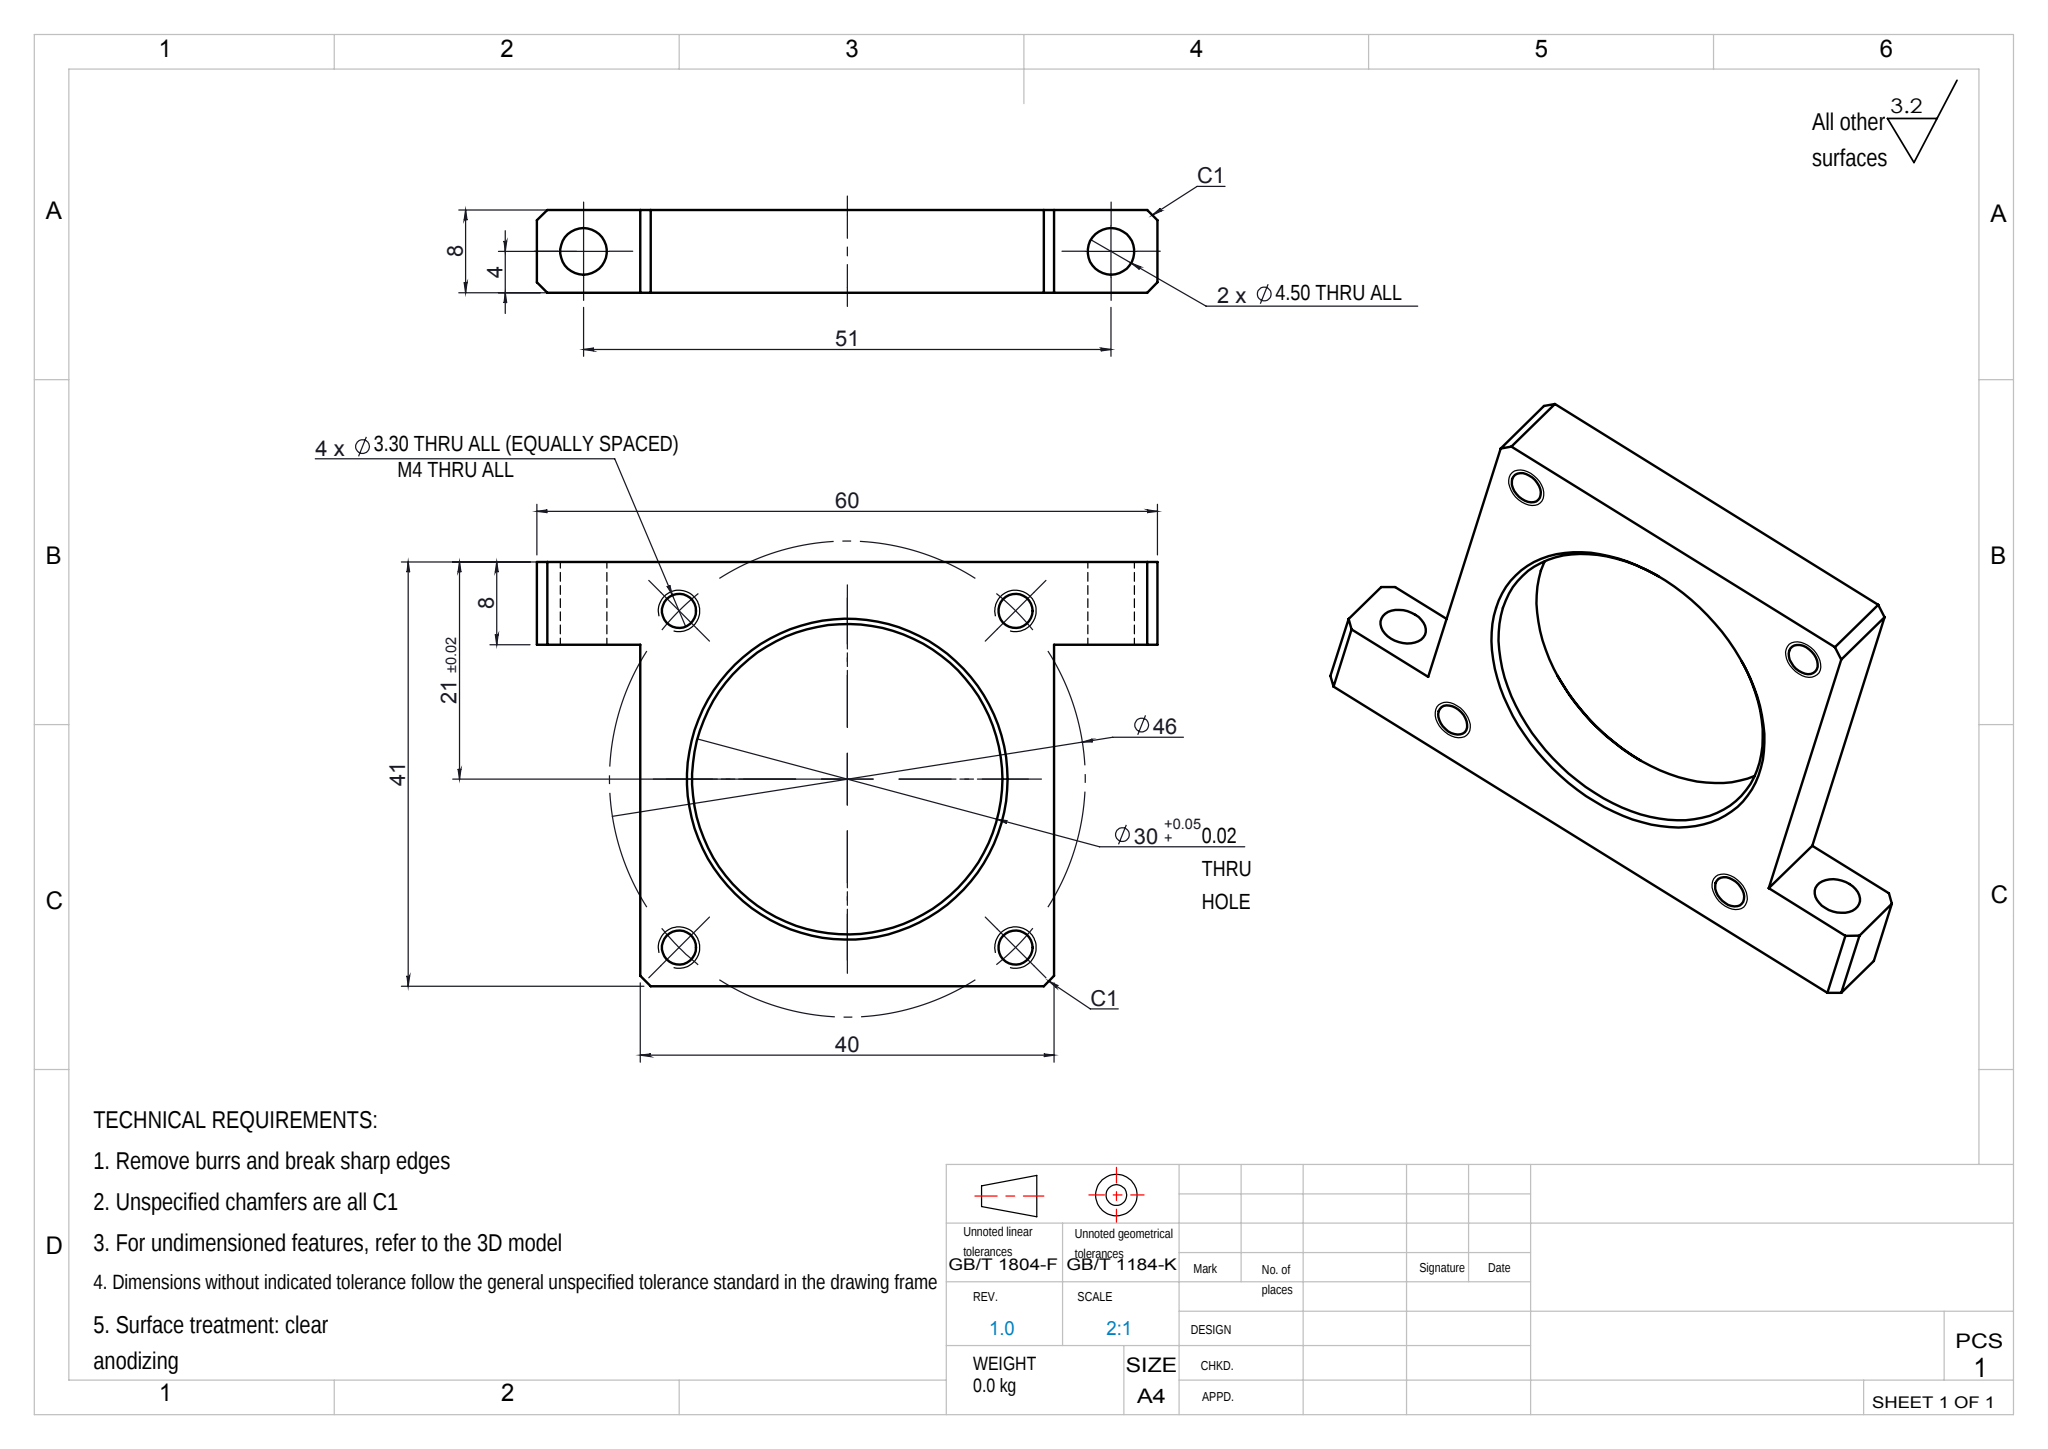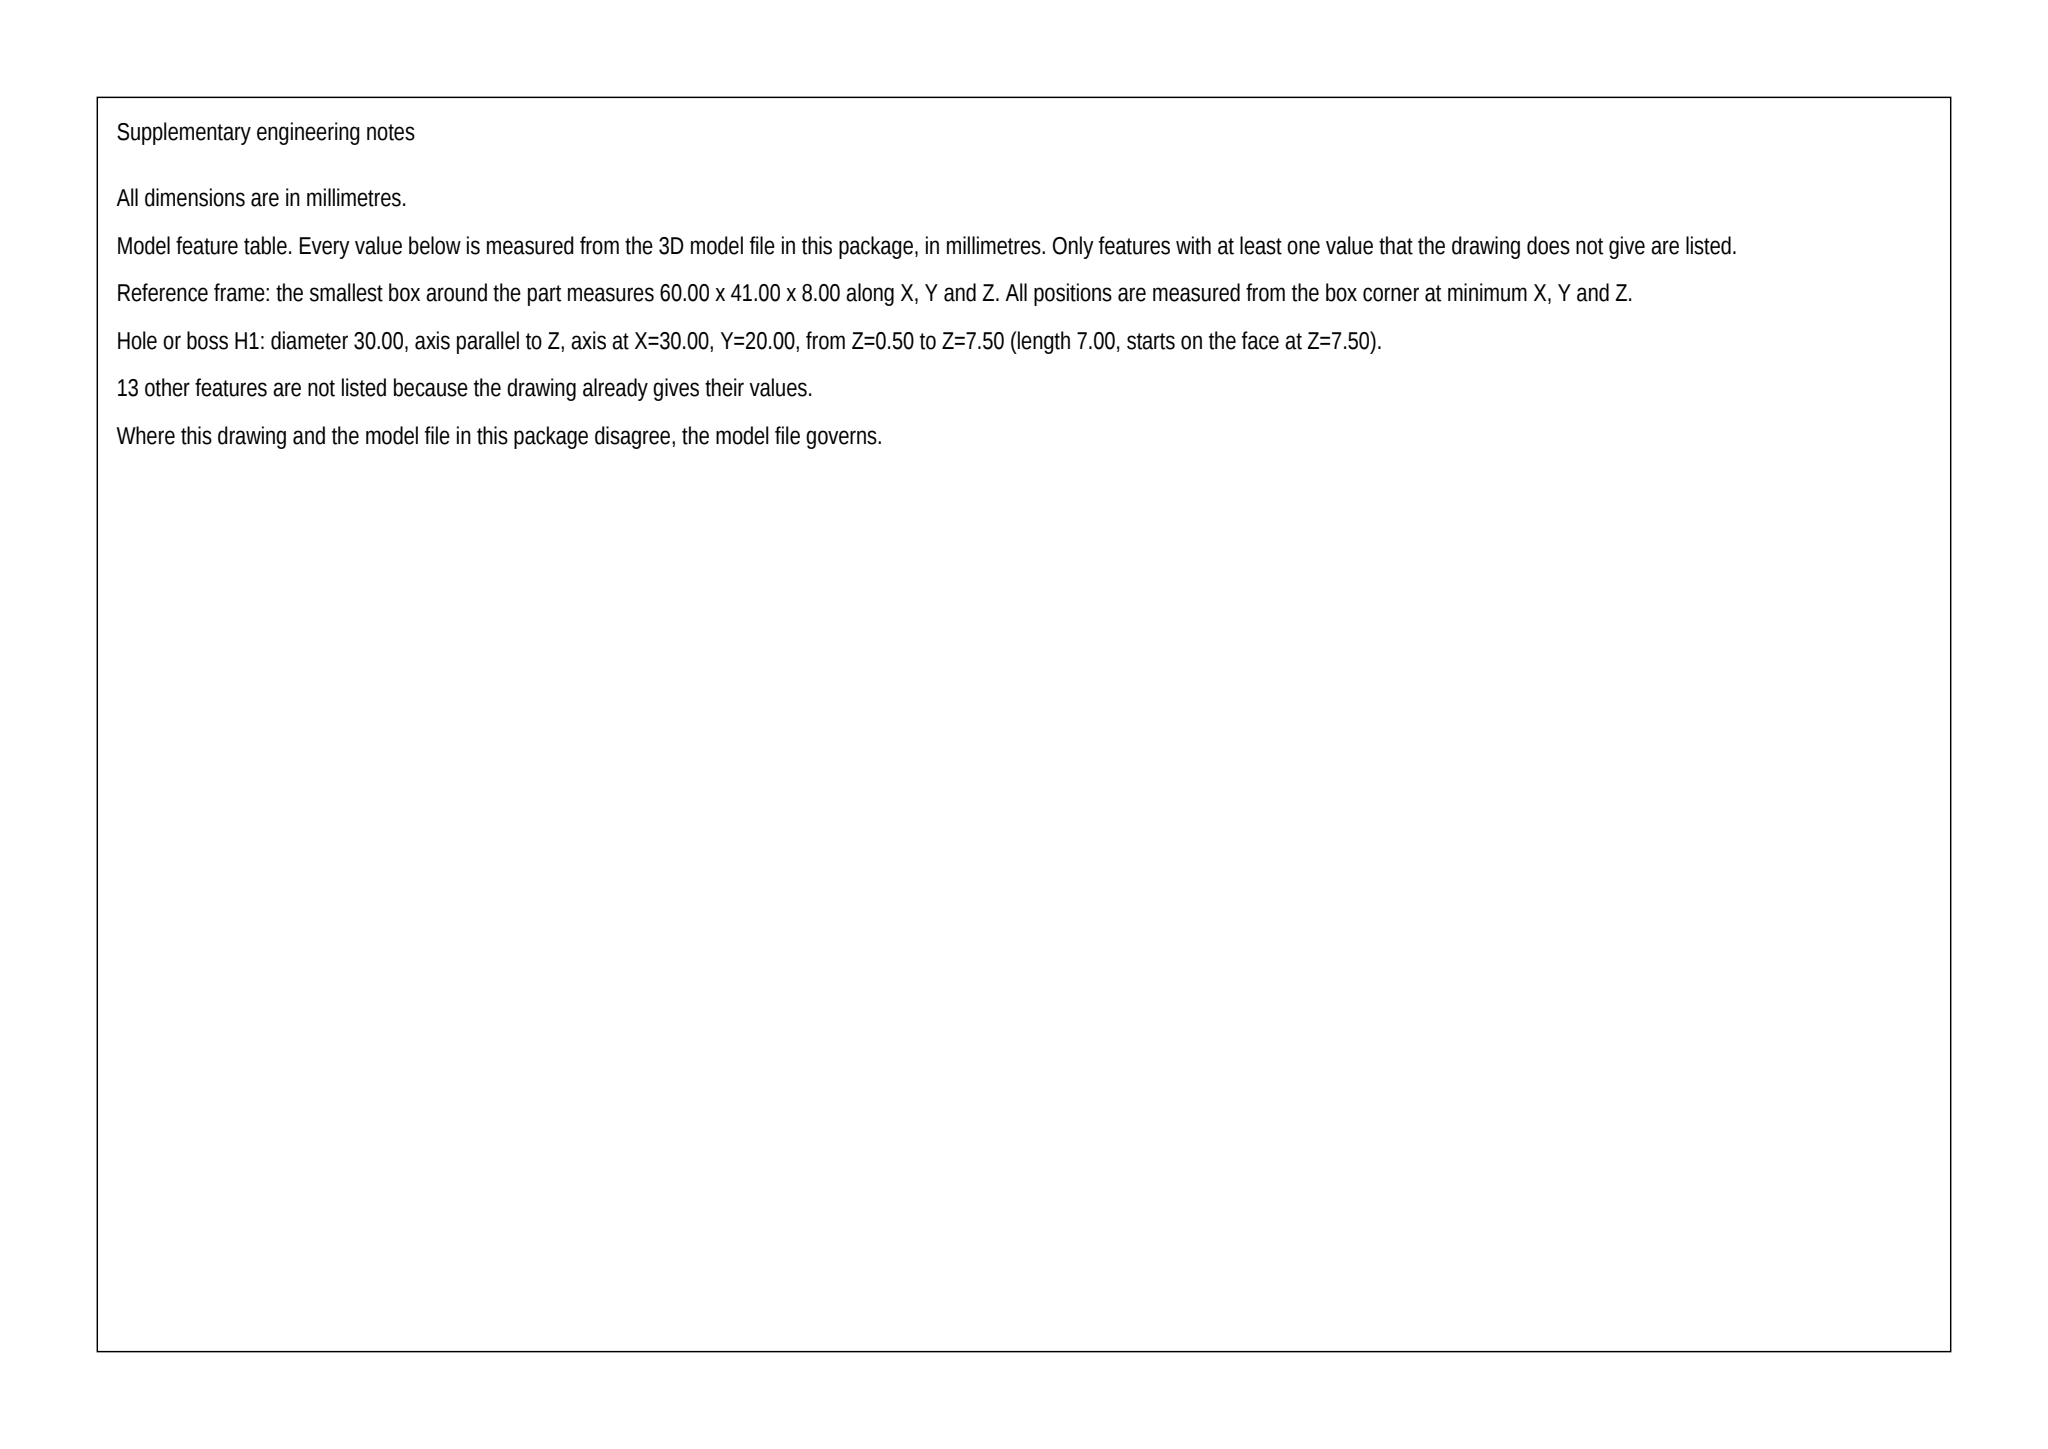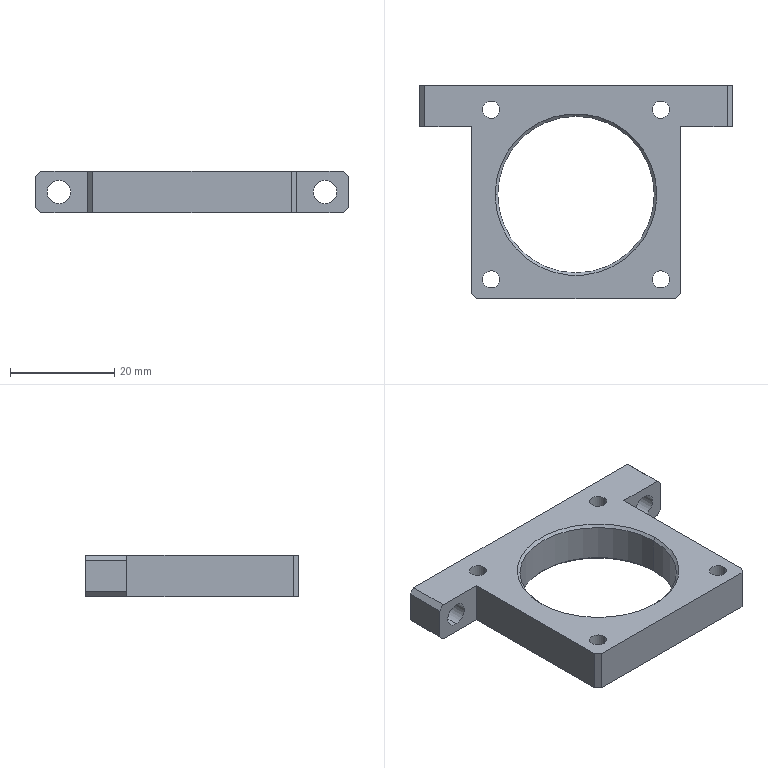Part | SolidWorks | mm | material AL 6061 | 1 solid | 34 faces | box 60 x 41 x 8 mm | volume 8169 mm3 | plane 16 | cylinder 14 | cone 4 | commonest cylinder face diameters 3.3 x8 4.5 x4 30 x2
Drawing notes:
4X Ø3.30 THRU, NO TAP - DISREGARD 'M4 THRU' | from the solid: 4 cylinders dia 3.30, axis z, from z0 to z8 at (13.7,3.7),(13.7,36.3),(46.3,3.7),(46.3,36.3); no thread geometry in STEP
CENTER BORE: Ø30.00 ±0.02 THRU, C0.5 BOTH ENDS | from the solid: cylinder dia 30.0 axis z at (30.0,20.0) from z0.5 to z7.5; 90deg cones ref dia 30/31 at each face = 0.5 chamfer
build123d program:
from build123d import *

# Parameters (mm, degrees)
SKETCH1_W            = 60
SKETCH1_H            = 41
BOSS_EXTRUDE1_DEPTH  = 8
SKETCH4_R            = 15
CUT_EXTRUDE2_DEPTH   = 38.206
M4_TAPPED_HOLE1_D    = 3.3
SKETCH23_W           = 10
SKETCH23_H           = 33
CUT_EXTRUDE3_DEPTH   = 38.206
M4_CLEARANCE_HOLE1_D = 4.5
CHAMFER2_SIZE        = 1
CHAMFER3_SIZE        = 0.5


with BuildPart() as part:
    # Sketch1 → Boss-Extrude1 (new body)
    with BuildSketch(Plane.XY):
        Rectangle(SKETCH1_W, SKETCH1_H)
    extrude(amount=BOSS_EXTRUDE1_DEPTH)

    # Sketch4 → Cut-Extrude2 (cut, through all)
    with BuildSketch(Plane.XY.offset(8)):
        with Locations((0, -0.5)):
            Circle(SKETCH4_R)
    extrude(amount=-CUT_EXTRUDE2_DEPTH, mode=Mode.SUBTRACT)

    # M4 Tapped Hole1 (through all)
    with Locations(Plane.XY.offset(8)):
        with Locations((-16.265, 15.763), (-16.265, -16.763), (16.265, 15.763), (16.265, -16.763)):
            Hole(M4_TAPPED_HOLE1_D / 2)

    # Sketch23 → Cut-Extrude3 (cut, through all)
    with BuildSketch(Plane.XY.offset(8)):
        with Locations((-25, -4)):
            Rectangle(SKETCH23_W, SKETCH23_H)
        with Locations((25, -4)):
            Rectangle(SKETCH23_W, SKETCH23_H)
    extrude(amount=-CUT_EXTRUDE3_DEPTH, mode=Mode.SUBTRACT)

    # M4 Clearance Hole1 (through all)
    with Locations(Plane(origin=(0, 12.5, 0), x_dir=(-1, 0, 0), z_dir=(0, -1, 0))):
        with Locations((25.5, -4), (-25.5, -4)):
            Hole(M4_CLEARANCE_HOLE1_D / 2)

    # Chamfer2
    chamfer2_edges = [part.edges().sort_by_distance(p)[0] for p in [
        (30, 16.5, 0),
        (30, 16.5, 8),
        (-30, 16.5, 8),
        (-20, -20.5, 4),
        (20, -20.5, 4),
        (-30, 16.5, 0),
    ]]
    chamfer(chamfer2_edges, length=CHAMFER2_SIZE)

    # Chamfer3
    chamfer3_edges = [part.edges().sort_by_distance(p)[0] for p in [
        (-15, -0.5, 0),
        (-15, -0.5, 8),
    ]]
    chamfer(chamfer3_edges, length=CHAMFER3_SIZE)


solid = part.part